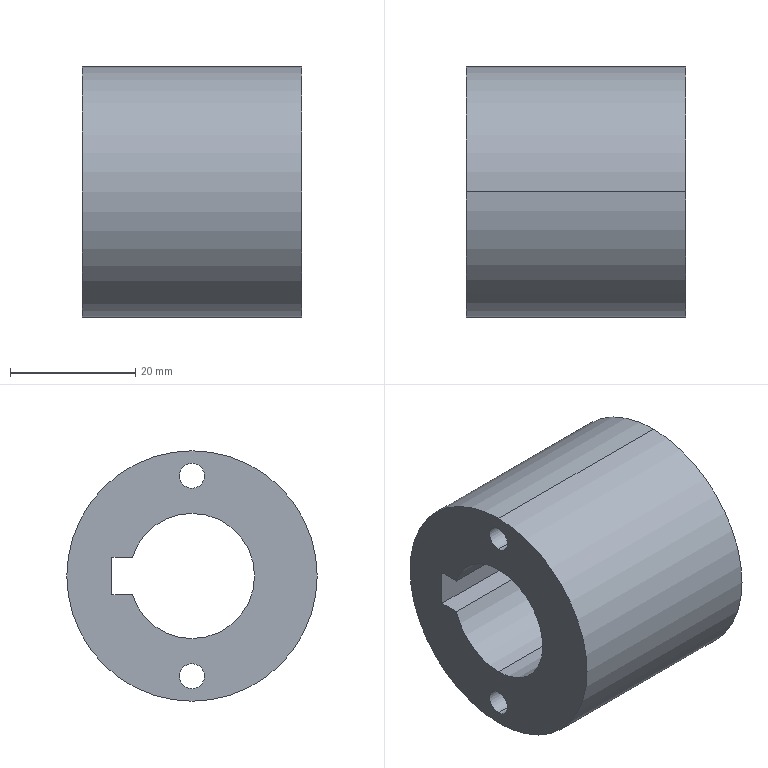Component | SolidWorks | CamGroup3-1_Cam8-1 | 1 solid | 14 faces | box 35 x 40 x 40 mm | volume 31490 mm3 | cylinder 9 | plane 5 | commonest cylinder face diameters 4 x4 20 x3 40 x2
build123d program:
from build123d import *

# Parameters (mm, degrees)
MODEL_R             = 20
MODEL_R_2           = 2
BOSS_EXTRUDE1_DEPTH = 35


with BuildPart() as part:
    # Model → Boss-Extrude1 (new body)
    with BuildSketch(Plane.XY):
        with Locations((103.927, 116.86)):
            Circle(MODEL_R)
        with Locations((87.927, 116.862)):
            Circle(MODEL_R_2, mode=Mode.SUBTRACT)
        with Locations((119.927, 116.862)):
            Circle(MODEL_R_2, mode=Mode.SUBTRACT)
        with BuildLine():
            Line((106.927, 129.646), (106.927, 126.401))
            ThreePointArc((106.927, 126.401), (103.927, 106.862), (100.927, 126.401))
            Line((100.927, 126.401), (100.927, 129.646))
            Line((100.927, 129.646), (106.927, 129.646))
        make_face(mode=Mode.SUBTRACT)
    extrude(amount=BOSS_EXTRUDE1_DEPTH)


solid = part.part

# Placed as in the assembly
solid = solid.moved(Location((-104.938, -101.746, 452.927), (0, 90, 0)))
STEP:
#1=COLOUR_RGB('',0.7922,0.8196,0.9333);
#2=FILL_AREA_STYLE_COLOUR('',#1);
#3=FILL_AREA_STYLE('',(#2));
#4=SURFACE_STYLE_FILL_AREA(#3);
#5=SURFACE_SIDE_STYLE('',(#4));
#6=SURFACE_STYLE_USAGE(.BOTH.,#5);
#7=PRESENTATION_STYLE_ASSIGNMENT((#6));
#8=CARTESIAN_POINT('',(-4.131,0.5951,13.346));
#9=VERTEX_POINT('',#8);
#10=CARTESIAN_POINT('',(-4.131,0.5951,14.134));
#11=VERTEX_POINT('',#10);
#12=CARTESIAN_POINT('',(-4.131,0.5951,13.74));
#13=DIRECTION('',(-1.,0.,0.));
#14=DIRECTION('',(0.,0.,1.));
#15=AXIS2_PLACEMENT_3D('',#12,#13,#14);
#16=CIRCLE('',#15,0.3937);
#17=EDGE_CURVE('',#9,#11,#16,.T.);
#18=ORIENTED_EDGE('',*,*,#17,.T.);
#19=CARTESIAN_POINT('',(-2.753,0.5951,14.134));
#20=VERTEX_POINT('',#19);
#21=CARTESIAN_POINT('',(-4.131,0.5951,14.134));
#22=DIRECTION('',(1.,0.,0.));
#23=VECTOR('',#22,39.37);
#24=LINE('',#21,#23);
#25=EDGE_CURVE('',#11,#20,#24,.T.);
#26=ORIENTED_EDGE('',*,*,#25,.T.);
#27=CARTESIAN_POINT('',(-2.753,0.5951,13.346));
#28=VERTEX_POINT('',#27);
#29=CARTESIAN_POINT('',(-2.753,0.5951,13.74));
#30=DIRECTION('',(-1.,0.,0.));
#31=DIRECTION('',(0.,0.,1.));
#32=AXIS2_PLACEMENT_3D('',#29,#30,#31);
#33=CIRCLE('',#32,0.3937);
#34=EDGE_CURVE('',#28,#20,#33,.T.);
#35=ORIENTED_EDGE('',*,*,#34,.F.);
#36=CARTESIAN_POINT('',(-4.131,0.5951,13.346));
#37=DIRECTION('',(1.,0.,0.));
#38=VECTOR('',#37,39.37);
#39=LINE('',#36,#38);
#40=EDGE_CURVE('',#9,#28,#39,.T.);
#41=ORIENTED_EDGE('',*,*,#40,.F.);
#42=EDGE_LOOP('',(#18,#26,#35,#41));
#43=FACE_OUTER_BOUND('',#42,.T.);
#44=CARTESIAN_POINT('',(-4.131,0.5951,13.74));
#45=DIRECTION('',(1.,0.,0.));
#46=DIRECTION('',(0.,-0.,-1.));
#47=AXIS2_PLACEMENT_3D('',#44,#45,#46);
#48=CYLINDRICAL_SURFACE('',#47,0.3937);
#49=ADVANCED_FACE('',(#43),#48,.F.);
#50=CARTESIAN_POINT('',(-4.131,0.9707,13.622));
#51=VERTEX_POINT('',#50);
#52=CARTESIAN_POINT('',(-4.131,0.5951,13.74));
#53=DIRECTION('',(-1.,0.,0.));
#54=DIRECTION('',(0.,0.,1.));
#55=AXIS2_PLACEMENT_3D('',#52,#53,#54);
#56=CIRCLE('',#55,0.3937);
#57=EDGE_CURVE('',#51,#9,#56,.T.);
#58=ORIENTED_EDGE('',*,*,#57,.T.);
#59=ORIENTED_EDGE('',*,*,#40,.T.);
#60=CARTESIAN_POINT('',(-2.753,0.9707,13.622));
#61=VERTEX_POINT('',#60);
#62=CARTESIAN_POINT('',(-2.753,0.5951,13.74));
#63=DIRECTION('',(-1.,0.,0.));
#64=DIRECTION('',(0.,0.,1.));
#65=AXIS2_PLACEMENT_3D('',#62,#63,#64);
#66=CIRCLE('',#65,0.3937);
#67=EDGE_CURVE('',#61,#28,#66,.T.);
#68=ORIENTED_EDGE('',*,*,#67,.F.);
#69=CARTESIAN_POINT('',(-4.131,0.9707,13.622));
#70=DIRECTION('',(1.,0.,0.));
#71=VECTOR('',#70,39.37);
#72=LINE('',#69,#71);
#73=EDGE_CURVE('',#51,#61,#72,.T.);
#74=ORIENTED_EDGE('',*,*,#73,.F.);
#75=EDGE_LOOP('',(#58,#59,#68,#74));
#76=FACE_OUTER_BOUND('',#75,.T.);
#77=CARTESIAN_POINT('',(-4.131,0.5951,13.74));
#78=DIRECTION('',(1.,0.,0.));
#79=DIRECTION('',(0.,-0.,-1.));
#80=AXIS2_PLACEMENT_3D('',#77,#78,#79);
#81=CYLINDRICAL_SURFACE('',#80,0.3937);
#82=ADVANCED_FACE('',(#76),#81,.F.);
#83=CARTESIAN_POINT('',(-4.131,0.5951,14.291));
#84=VERTEX_POINT('',#83);
#85=CARTESIAN_POINT('',(-4.131,0.5951,14.449));
#86=VERTEX_POINT('',#85);
#87=CARTESIAN_POINT('',(-4.131,0.5951,14.37));
#88=DIRECTION('',(-1.,0.,0.));
#89=DIRECTION('',(0.,0.,1.));
#90=AXIS2_PLACEMENT_3D('',#87,#88,#89);
#91=CIRCLE('',#90,0.07874);
#92=EDGE_CURVE('',#84,#86,#91,.T.);
#93=ORIENTED_EDGE('',*,*,#92,.T.);
#94=CARTESIAN_POINT('',(-2.753,0.5951,14.449));
#95=VERTEX_POINT('',#94);
#96=CARTESIAN_POINT('',(-4.131,0.5951,14.449));
#97=DIRECTION('',(1.,0.,0.));
#98=VECTOR('',#97,39.37);
#99=LINE('',#96,#98);
#100=EDGE_CURVE('',#86,#95,#99,.T.);
#101=ORIENTED_EDGE('',*,*,#100,.T.);
#102=CARTESIAN_POINT('',(-2.753,0.5951,14.291));
#103=VERTEX_POINT('',#102);
#104=CARTESIAN_POINT('',(-2.753,0.5951,14.37));
#105=DIRECTION('',(-1.,0.,0.));
#106=DIRECTION('',(0.,0.,1.));
#107=AXIS2_PLACEMENT_3D('',#104,#105,#106);
#108=CIRCLE('',#107,0.07874);
#109=EDGE_CURVE('',#103,#95,#108,.T.);
#110=ORIENTED_EDGE('',*,*,#109,.F.);
#111=CARTESIAN_POINT('',(-4.131,0.5951,14.291));
#112=DIRECTION('',(1.,0.,0.));
#113=VECTOR('',#112,39.37);
#114=LINE('',#111,#113);
#115=EDGE_CURVE('',#84,#103,#114,.T.);
#116=ORIENTED_EDGE('',*,*,#115,.F.);
#117=EDGE_LOOP('',(#93,#101,#110,#116));
#118=FACE_OUTER_BOUND('',#117,.T.);
#119=CARTESIAN_POINT('',(-4.131,0.5951,14.37));
#120=DIRECTION('',(1.,0.,0.));
#121=DIRECTION('',(0.,0.,-1.));
#122=AXIS2_PLACEMENT_3D('',#119,#120,#121);
#123=CYLINDRICAL_SURFACE('',#122,0.07874);
#124=ADVANCED_FACE('',(#118),#123,.F.);
#125=CARTESIAN_POINT('',(-4.131,0.5951,13.031));
#126=VERTEX_POINT('',#125);
#127=CARTESIAN_POINT('',(-4.131,0.5951,13.189));
#128=VERTEX_POINT('',#127);
#129=CARTESIAN_POINT('',(-4.131,0.5951,13.11));
#130=DIRECTION('',(-1.,0.,0.));
#131=DIRECTION('',(0.,0.,1.));
#132=AXIS2_PLACEMENT_3D('',#129,#130,#131);
#133=CIRCLE('',#132,0.07874);
#134=EDGE_CURVE('',#126,#128,#133,.T.);
#135=ORIENTED_EDGE('',*,*,#134,.T.);
#136=CARTESIAN_POINT('',(-2.753,0.5951,13.189));
#137=VERTEX_POINT('',#136);
#138=CARTESIAN_POINT('',(-4.131,0.5951,13.189));
#139=DIRECTION('',(1.,0.,0.));
#140=VECTOR('',#139,39.37);
#141=LINE('',#138,#140);
#142=EDGE_CURVE('',#128,#137,#141,.T.);
#143=ORIENTED_EDGE('',*,*,#142,.T.);
#144=CARTESIAN_POINT('',(-2.753,0.5951,13.031));
#145=VERTEX_POINT('',#144);
#146=CARTESIAN_POINT('',(-2.753,0.5951,13.11));
#147=DIRECTION('',(-1.,0.,0.));
#148=DIRECTION('',(0.,0.,1.));
#149=AXIS2_PLACEMENT_3D('',#146,#147,#148);
#150=CIRCLE('',#149,0.07874);
#151=EDGE_CURVE('',#145,#137,#150,.T.);
#152=ORIENTED_EDGE('',*,*,#151,.F.);
#153=CARTESIAN_POINT('',(-4.131,0.5951,13.031));
#154=DIRECTION('',(1.,0.,0.));
#155=VECTOR('',#154,39.37);
#156=LINE('',#153,#155);
#157=EDGE_CURVE('',#126,#145,#156,.T.);
#158=ORIENTED_EDGE('',*,*,#157,.F.);
#159=EDGE_LOOP('',(#135,#143,#152,#158));
#160=FACE_OUTER_BOUND('',#159,.T.);
#161=CARTESIAN_POINT('',(-4.131,0.5951,13.11));
#162=DIRECTION('',(1.,0.,0.));
#163=DIRECTION('',(0.,0.,-1.));
#164=AXIS2_PLACEMENT_3D('',#161,#162,#163);
#165=CYLINDRICAL_SURFACE('',#164,0.07874);
#166=ADVANCED_FACE('',(#160),#165,.F.);
#167=CARTESIAN_POINT('',(-4.131,0.595,14.528));
#168=VERTEX_POINT('',#167);
#169=CARTESIAN_POINT('',(-4.131,0.595,12.953));
#170=VERTEX_POINT('',#169);
#171=CARTESIAN_POINT('',(-4.131,0.595,13.74));
#172=DIRECTION('',(-1.,0.,0.));
#173=DIRECTION('',(0.,0.,1.));
#174=AXIS2_PLACEMENT_3D('',#171,#172,#173);
#175=CIRCLE('',#174,0.7874);
#176=EDGE_CURVE('',#168,#170,#175,.T.);
#177=ORIENTED_EDGE('',*,*,#176,.F.);
#178=CARTESIAN_POINT('',(-2.753,0.595,14.528));
#179=VERTEX_POINT('',#178);
#180=CARTESIAN_POINT('',(-4.131,0.595,14.528));
#181=DIRECTION('',(1.,0.,0.));
#182=VECTOR('',#181,39.37);
#183=LINE('',#180,#182);
#184=EDGE_CURVE('',#168,#179,#183,.T.);
#185=ORIENTED_EDGE('',*,*,#184,.T.);
#186=CARTESIAN_POINT('',(-2.753,0.595,12.953));
#187=VERTEX_POINT('',#186);
#188=CARTESIAN_POINT('',(-2.753,0.595,13.74));
#189=DIRECTION('',(-1.,0.,0.));
#190=DIRECTION('',(0.,0.,1.));
#191=AXIS2_PLACEMENT_3D('',#188,#189,#190);
#192=CIRCLE('',#191,0.7874);
#193=EDGE_CURVE('',#179,#187,#192,.T.);
#194=ORIENTED_EDGE('',*,*,#193,.T.);
#195=CARTESIAN_POINT('',(-4.131,0.595,12.953));
#196=DIRECTION('',(1.,0.,0.));
#197=VECTOR('',#196,39.37);
#198=LINE('',#195,#197);
#199=EDGE_CURVE('',#170,#187,#198,.T.);
#200=ORIENTED_EDGE('',*,*,#199,.F.);
#201=EDGE_LOOP('',(#177,#185,#194,#200));
#202=FACE_OUTER_BOUND('',#201,.T.);
#203=CARTESIAN_POINT('',(-4.131,0.595,13.74));
#204=DIRECTION('',(1.,0.,0.));
#205=DIRECTION('',(0.,-0.,-1.));
#206=AXIS2_PLACEMENT_3D('',#203,#204,#205);
#207=CYLINDRICAL_SURFACE('',#206,0.7874);
#208=ADVANCED_FACE('',(#202),#207,.T.);
#209=ORIENTED_EDGE('',*,*,#134,.F.);
#210=CARTESIAN_POINT('',(-4.131,0.5951,13.11));
#211=DIRECTION('',(-1.,0.,0.));
#212=DIRECTION('',(0.,0.,1.));
#213=AXIS2_PLACEMENT_3D('',#210,#211,#212);
#214=CIRCLE('',#213,0.07874);
#215=EDGE_CURVE('',#128,#126,#214,.T.);
#216=ORIENTED_EDGE('',*,*,#215,.F.);
#217=EDGE_LOOP('',(#209,#216));
#218=FACE_BOUND('',#217,.T.);
#219=CARTESIAN_POINT('',(-4.131,0.595,13.74));
#220=DIRECTION('',(-1.,0.,0.));
#221=DIRECTION('',(0.,0.,1.));
#222=AXIS2_PLACEMENT_3D('',#219,#220,#221);
#223=CIRCLE('',#222,0.7874);
#224=EDGE_CURVE('',#170,#168,#223,.T.);
#225=ORIENTED_EDGE('',*,*,#224,.T.);
#226=ORIENTED_EDGE('',*,*,#176,.T.);
#227=EDGE_LOOP('',(#225,#226));
#228=FACE_OUTER_BOUND('',#227,.T.);
#229=ORIENTED_EDGE('',*,*,#92,.F.);
#230=CARTESIAN_POINT('',(-4.131,0.5951,14.37));
#231=DIRECTION('',(-1.,0.,0.));
#232=DIRECTION('',(0.,0.,1.));
#233=AXIS2_PLACEMENT_3D('',#230,#231,#232);
#234=CIRCLE('',#233,0.07874);
#235=EDGE_CURVE('',#86,#84,#234,.T.);
#236=ORIENTED_EDGE('',*,*,#235,.F.);
#237=EDGE_LOOP('',(#229,#236));
#238=FACE_BOUND('',#237,.T.);
#239=CARTESIAN_POINT('',(-4.131,0.9707,13.858));
#240=VERTEX_POINT('',#239);
#241=CARTESIAN_POINT('',(-4.131,1.098,13.858));
#242=VERTEX_POINT('',#241);
#243=CARTESIAN_POINT('',(-4.131,1.098,13.858));
#244=DIRECTION('',(0.,1.,-0.));
#245=VECTOR('',#244,39.37);
#246=LINE('',#243,#245);
#247=EDGE_CURVE('',#240,#242,#246,.T.);
#248=ORIENTED_EDGE('',*,*,#247,.F.);
#249=CARTESIAN_POINT('',(-4.131,0.5951,13.74));
#250=DIRECTION('',(-1.,0.,0.));
#251=DIRECTION('',(0.,0.,1.));
#252=AXIS2_PLACEMENT_3D('',#249,#250,#251);
#253=CIRCLE('',#252,0.3937);
#254=EDGE_CURVE('',#11,#240,#253,.T.);
#255=ORIENTED_EDGE('',*,*,#254,.F.);
#256=ORIENTED_EDGE('',*,*,#17,.F.);
#257=ORIENTED_EDGE('',*,*,#57,.F.);
#258=CARTESIAN_POINT('',(-4.131,1.098,13.622));
#259=VERTEX_POINT('',#258);
#260=CARTESIAN_POINT('',(-4.131,1.098,13.622));
#261=DIRECTION('',(0.,-1.,0.));
#262=VECTOR('',#261,39.37);
#263=LINE('',#260,#262);
#264=EDGE_CURVE('',#259,#51,#263,.T.);
#265=ORIENTED_EDGE('',*,*,#264,.F.);
#266=CARTESIAN_POINT('',(-4.131,1.098,13.858));
#267=DIRECTION('',(0.,-0.,-1.));
#268=VECTOR('',#267,39.37);
#269=LINE('',#266,#268);
#270=EDGE_CURVE('',#242,#259,#269,.T.);
#271=ORIENTED_EDGE('',*,*,#270,.F.);
#272=EDGE_LOOP('',(#248,#255,#256,#257,#265,#271));
#273=FACE_BOUND('',#272,.T.);
#274=CARTESIAN_POINT('',(-4.131,0.595,13.74));
#275=DIRECTION('',(-1.,0.,0.));
#276=DIRECTION('',(0.,0.,1.));
#277=AXIS2_PLACEMENT_3D('',#274,#275,#276);
#278=PLANE('',#277);
#279=ADVANCED_FACE('',(#218,#228,#238,#273),#278,.T.);
#280=ORIENTED_EDGE('',*,*,#109,.T.);
#281=CARTESIAN_POINT('',(-2.753,0.5951,14.37));
#282=DIRECTION('',(-1.,0.,0.));
#283=DIRECTION('',(0.,0.,1.));
#284=AXIS2_PLACEMENT_3D('',#281,#282,#283);
#285=CIRCLE('',#284,0.07874);
#286=EDGE_CURVE('',#95,#103,#285,.T.);
#287=ORIENTED_EDGE('',*,*,#286,.T.);
#288=EDGE_LOOP('',(#280,#287));
#289=FACE_BOUND('',#288,.T.);
#290=ORIENTED_EDGE('',*,*,#151,.T.);
#291=CARTESIAN_POINT('',(-2.753,0.5951,13.11));
#292=DIRECTION('',(-1.,0.,0.));
#293=DIRECTION('',(0.,0.,1.));
#294=AXIS2_PLACEMENT_3D('',#291,#292,#293);
#295=CIRCLE('',#294,0.07874);
#296=EDGE_CURVE('',#137,#145,#295,.T.);
#297=ORIENTED_EDGE('',*,*,#296,.T.);
#298=EDGE_LOOP('',(#290,#297));
#299=FACE_BOUND('',#298,.T.);
#300=CARTESIAN_POINT('',(-2.753,0.595,13.74));
#301=DIRECTION('',(-1.,0.,0.));
#302=DIRECTION('',(0.,0.,1.));
#303=AXIS2_PLACEMENT_3D('',#300,#301,#302);
#304=CIRCLE('',#303,0.7874);
#305=EDGE_CURVE('',#187,#179,#304,.T.);
#306=ORIENTED_EDGE('',*,*,#305,.F.);
#307=ORIENTED_EDGE('',*,*,#193,.F.);
#308=EDGE_LOOP('',(#306,#307));
#309=FACE_OUTER_BOUND('',#308,.T.);
#310=ORIENTED_EDGE('',*,*,#67,.T.);
#311=ORIENTED_EDGE('',*,*,#34,.T.);
#312=CARTESIAN_POINT('',(-2.753,0.9707,13.858));
#313=VERTEX_POINT('',#312);
#314=CARTESIAN_POINT('',(-2.753,0.5951,13.74));
#315=DIRECTION('',(-1.,0.,0.));
#316=DIRECTION('',(0.,0.,1.));
#317=AXIS2_PLACEMENT_3D('',#314,#315,#316);
#318=CIRCLE('',#317,0.3937);
#319=EDGE_CURVE('',#20,#313,#318,.T.);
#320=ORIENTED_EDGE('',*,*,#319,.T.);
#321=CARTESIAN_POINT('',(-2.753,1.098,13.858));
#322=VERTEX_POINT('',#321);
#323=CARTESIAN_POINT('',(-2.753,1.098,13.858));
#324=DIRECTION('',(0.,1.,-0.));
#325=VECTOR('',#324,39.37);
#326=LINE('',#323,#325);
#327=EDGE_CURVE('',#313,#322,#326,.T.);
#328=ORIENTED_EDGE('',*,*,#327,.T.);
#329=CARTESIAN_POINT('',(-2.753,1.098,13.622));
#330=VERTEX_POINT('',#329);
#331=CARTESIAN_POINT('',(-2.753,1.098,13.858));
#332=DIRECTION('',(0.,-0.,-1.));
#333=VECTOR('',#332,39.37);
#334=LINE('',#331,#333);
#335=EDGE_CURVE('',#322,#330,#334,.T.);
#336=ORIENTED_EDGE('',*,*,#335,.T.);
#337=CARTESIAN_POINT('',(-2.753,1.098,13.622));
#338=DIRECTION('',(0.,-1.,0.));
#339=VECTOR('',#338,39.37);
#340=LINE('',#337,#339);
#341=EDGE_CURVE('',#330,#61,#340,.T.);
#342=ORIENTED_EDGE('',*,*,#341,.T.);
#343=EDGE_LOOP('',(#310,#311,#320,#328,#336,#342));
#344=FACE_BOUND('',#343,.T.);
#345=CARTESIAN_POINT('',(-2.753,0.595,13.74));
#346=DIRECTION('',(-1.,0.,0.));
#347=DIRECTION('',(0.,0.,1.));
#348=AXIS2_PLACEMENT_3D('',#345,#346,#347);
#349=PLANE('',#348);
#350=ADVANCED_FACE('',(#289,#299,#309,#344),#349,.F.);
#351=ORIENTED_EDGE('',*,*,#184,.F.);
#352=ORIENTED_EDGE('',*,*,#224,.F.);
#353=ORIENTED_EDGE('',*,*,#199,.T.);
#354=ORIENTED_EDGE('',*,*,#305,.T.);
#355=EDGE_LOOP('',(#351,#352,#353,#354));
#356=FACE_OUTER_BOUND('',#355,.T.);
#357=CARTESIAN_POINT('',(-4.131,0.595,13.74));
#358=DIRECTION('',(1.,0.,0.));
#359=DIRECTION('',(0.,-0.,-1.));
#360=AXIS2_PLACEMENT_3D('',#357,#358,#359);
#361=CYLINDRICAL_SURFACE('',#360,0.7874);
#362=ADVANCED_FACE('',(#356),#361,.T.);
#363=ORIENTED_EDGE('',*,*,#142,.F.);
#364=ORIENTED_EDGE('',*,*,#215,.T.);
#365=ORIENTED_EDGE('',*,*,#157,.T.);
#366=ORIENTED_EDGE('',*,*,#296,.F.);
#367=EDGE_LOOP('',(#363,#364,#365,#366));
#368=FACE_OUTER_BOUND('',#367,.T.);
#369=CARTESIAN_POINT('',(-4.131,0.5951,13.11));
#370=DIRECTION('',(1.,0.,0.));
#371=DIRECTION('',(0.,0.,-1.));
#372=AXIS2_PLACEMENT_3D('',#369,#370,#371);
#373=CYLINDRICAL_SURFACE('',#372,0.07874);
#374=ADVANCED_FACE('',(#368),#373,.F.);
#375=ORIENTED_EDGE('',*,*,#100,.F.);
#376=ORIENTED_EDGE('',*,*,#235,.T.);
#377=ORIENTED_EDGE('',*,*,#115,.T.);
#378=ORIENTED_EDGE('',*,*,#286,.F.);
#379=EDGE_LOOP('',(#375,#376,#377,#378));
#380=FACE_OUTER_BOUND('',#379,.T.);
#381=CARTESIAN_POINT('',(-4.131,0.5951,14.37));
#382=DIRECTION('',(1.,0.,0.));
#383=DIRECTION('',(0.,0.,-1.));
#384=AXIS2_PLACEMENT_3D('',#381,#382,#383);
#385=CYLINDRICAL_SURFACE('',#384,0.07874);
#386=ADVANCED_FACE('',(#380),#385,.F.);
#387=ORIENTED_EDGE('',*,*,#25,.F.);
#388=ORIENTED_EDGE('',*,*,#254,.T.);
#389=CARTESIAN_POINT('',(-4.131,0.9707,13.858));
#390=DIRECTION('',(1.,0.,0.));
#391=VECTOR('',#390,39.37);
#392=LINE('',#389,#391);
#393=EDGE_CURVE('',#240,#313,#392,.T.);
#394=ORIENTED_EDGE('',*,*,#393,.T.);
#395=ORIENTED_EDGE('',*,*,#319,.F.);
#396=EDGE_LOOP('',(#387,#388,#394,#395));
#397=FACE_OUTER_BOUND('',#396,.T.);
#398=CARTESIAN_POINT('',(-4.131,0.5951,13.74));
#399=DIRECTION('',(1.,0.,0.));
#400=DIRECTION('',(0.,-0.,-1.));
#401=AXIS2_PLACEMENT_3D('',#398,#399,#400);
#402=CYLINDRICAL_SURFACE('',#401,0.3937);
#403=ADVANCED_FACE('',(#397),#402,.F.);
#404=ORIENTED_EDGE('',*,*,#327,.F.);
#405=ORIENTED_EDGE('',*,*,#393,.F.);
#406=ORIENTED_EDGE('',*,*,#247,.T.);
#407=CARTESIAN_POINT('',(-4.131,1.098,13.858));
#408=DIRECTION('',(1.,0.,0.));
#409=VECTOR('',#408,39.37);
#410=LINE('',#407,#409);
#411=EDGE_CURVE('',#242,#322,#410,.T.);
#412=ORIENTED_EDGE('',*,*,#411,.T.);
#413=EDGE_LOOP('',(#404,#405,#406,#412));
#414=FACE_OUTER_BOUND('',#413,.T.);
#415=CARTESIAN_POINT('',(-4.131,1.098,13.858));
#416=DIRECTION('',(0.,-0.,-1.));
#417=DIRECTION('',(-1.,0.,0.));
#418=AXIS2_PLACEMENT_3D('',#415,#416,#417);
#419=PLANE('',#418);
#420=ADVANCED_FACE('',(#414),#419,.T.);
#421=ORIENTED_EDGE('',*,*,#335,.F.);
#422=ORIENTED_EDGE('',*,*,#411,.F.);
#423=ORIENTED_EDGE('',*,*,#270,.T.);
#424=CARTESIAN_POINT('',(-4.131,1.098,13.622));
#425=DIRECTION('',(1.,0.,0.));
#426=VECTOR('',#425,39.37);
#427=LINE('',#424,#426);
#428=EDGE_CURVE('',#259,#330,#427,.T.);
#429=ORIENTED_EDGE('',*,*,#428,.T.);
#430=EDGE_LOOP('',(#421,#422,#423,#429));
#431=FACE_OUTER_BOUND('',#430,.T.);
#432=CARTESIAN_POINT('',(-4.131,1.098,13.858));
#433=DIRECTION('',(0.,-1.,0.));
#434=DIRECTION('',(1.,0.,0.));
#435=AXIS2_PLACEMENT_3D('',#432,#433,#434);
#436=PLANE('',#435);
#437=ADVANCED_FACE('',(#431),#436,.T.);
#438=ORIENTED_EDGE('',*,*,#341,.F.);
#439=ORIENTED_EDGE('',*,*,#428,.F.);
#440=ORIENTED_EDGE('',*,*,#264,.T.);
#441=ORIENTED_EDGE('',*,*,#73,.T.);
#442=EDGE_LOOP('',(#438,#439,#440,#441));
#443=FACE_OUTER_BOUND('',#442,.T.);
#444=CARTESIAN_POINT('',(-4.131,1.098,13.622));
#445=DIRECTION('',(0.,0.,1.));
#446=DIRECTION('',(1.,0.,0.));
#447=AXIS2_PLACEMENT_3D('',#444,#445,#446);
#448=PLANE('',#447);
#449=ADVANCED_FACE('',(#443),#448,.T.);
#450=CLOSED_SHELL('',(#49,#82,#124,#166,#208,#279,#350,#362,#374,#386,#403,#420,#437,#449));
#451=MANIFOLD_SOLID_BREP('',#450);
#452=STYLED_ITEM('',(#7),#451);
#453=(LENGTH_UNIT()NAMED_UNIT(*)SI_UNIT($,.METRE.));
#454=LENGTH_MEASURE_WITH_UNIT(LENGTH_MEASURE(0.0254),#453);
#455=DIMENSIONAL_EXPONENTS(1.,0.,0.,0.,0.,0.,0.);
#456=(CONVERSION_BASED_UNIT('',#454)LENGTH_UNIT()NAMED_UNIT(#455));
#457=UNCERTAINTY_MEASURE_WITH_UNIT(LENGTH_MEASURE(0.00001),#456,'','');
#458=(NAMED_UNIT(*)PLANE_ANGLE_UNIT()SI_UNIT($,.RADIAN.));
#459=(NAMED_UNIT(*)SI_UNIT($,.STERADIAN.)SOLID_ANGLE_UNIT());
#460=(GEOMETRIC_REPRESENTATION_CONTEXT(3)GLOBAL_UNCERTAINTY_ASSIGNED_CONTEXT((#457))GLOBAL_UNIT_ASSIGNED_CONTEXT((#456,#458,#459))REPRESENTATION_CONTEXT('',''));
#461=MECHANICAL_DESIGN_GEOMETRIC_PRESENTATION_REPRESENTATION('',(#452),#460);
#462=CARTESIAN_POINT('',(0.,0.,0.));
#463=DIRECTION('',(0.,0.,1.));
#464=DIRECTION('',(1.,0.,0.));
#465=AXIS2_PLACEMENT_3D('',#462,#463,#464);
#466=(LENGTH_UNIT()NAMED_UNIT(*)SI_UNIT($,.METRE.));
#467=LENGTH_MEASURE_WITH_UNIT(LENGTH_MEASURE(0.0254),#466);
#468=DIMENSIONAL_EXPONENTS(1.,0.,0.,0.,0.,0.,0.);
#469=(CONVERSION_BASED_UNIT('',#467)LENGTH_UNIT()NAMED_UNIT(#468));
#470=UNCERTAINTY_MEASURE_WITH_UNIT(LENGTH_MEASURE(0.00001),#469,'','');
#471=(NAMED_UNIT(*)PLANE_ANGLE_UNIT()SI_UNIT($,.RADIAN.));
#472=(NAMED_UNIT(*)SI_UNIT($,.STERADIAN.)SOLID_ANGLE_UNIT());
#473=(GEOMETRIC_REPRESENTATION_CONTEXT(3)GLOBAL_UNCERTAINTY_ASSIGNED_CONTEXT((#470))GLOBAL_UNIT_ASSIGNED_CONTEXT((#469,#471,#472))REPRESENTATION_CONTEXT('',''));
#474=ADVANCED_BREP_SHAPE_REPRESENTATION('',(#451,#465),#473);
#475=PRESENTATION_LAYER_ASSIGNMENT('','',(#452));